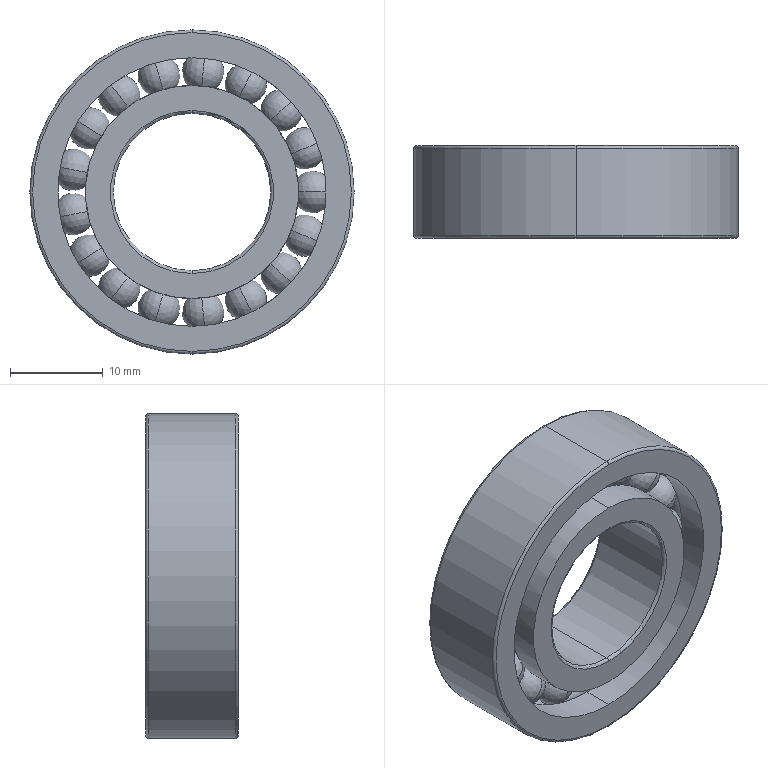Component | SolidWorks | -6003-1 | 1 solid | 112 faces | box 35 x 10 x 35 mm | volume 5427 mm3 | torus 62 | sphere 34 | cylinder 12 | plane 4 | commonest cylinder face diameters 29 x4 23 x4 35 x2 17 x2
build123d program:
from build123d import *

# Parameters (mm, degrees)
CIRCULAR_PATTERN1_COUNT = 17
FILLET1_R               = 0.3


with BuildPart() as part:
    # Sketch1 → Revolve1 (revolve)
    with BuildSketch(Plane.XY):
        with BuildLine():
            Line((-2.25, 13), (2.25, 13))
            ThreePointArc((2.25, 13), (0, 15.25), (-2.25, 13))
        make_face()
    revolve1 = revolve(axis=Axis((-4.597, 13, 0), (1, 0, 0)))

    # Sketch2 → Revolve2 (revolve)
    with BuildSketch(Plane.XY, mode=Mode.PRIVATE) as revolve2_sk:
        with BuildLine():
            Line((-5, 11.5), (-5, 8.5))
            Line((-5, 8.5), (5, 8.5))
            Line((5, 8.5), (5, 11.5))
            Line((5, 11.5), (1.664, 11.5))
            ThreePointArc((1.664, 11.5), (0, 10.76), (-1.664, 11.5))
            Line((-1.664, 11.5), (-5, 11.5))
        make_face()
    revolve(revolve2_sk.sketch.rotate(Axis((-6.971, 0, 0), (1, 0, 0)), 90), axis=Axis((-6.971, 0, 0), (1, 0, 0)))

    # Sketch3 → Revolve3 (revolve)
    with BuildSketch(Plane.XY, mode=Mode.PRIVATE) as revolve3_sk:
        with BuildLine():
            Line((-5, 17.5), (5, 17.5))
            Line((5, 17.5), (5, 14.5))
            Line((5, 14.5), (1.664, 14.5))
            ThreePointArc((1.664, 14.5), (0, 15.24), (-1.664, 14.5))
            Line((-1.664, 14.5), (-5, 14.5))
            Line((-5, 14.5), (-5, 17.5))
        make_face()
    revolve(revolve3_sk.sketch.rotate(Axis((-8.711, 0, 0), (1, 0, 0)), 90), axis=Axis((-8.711, 0, 0), (1, 0, 0)))

    # Circular-Pattern1: Revolve1 ×17 about axis
    circular_pattern1_axis = Axis((0, 0, 0), (1, 0, 0))
    for i in range(1, CIRCULAR_PATTERN1_COUNT):
        add(revolve1.rotate(circular_pattern1_axis, i * 360 / CIRCULAR_PATTERN1_COUNT))

    # Fillet1
    fillet1_edges = [part.edges().sort_by_distance(p)[0] for p in [
        (-5, 0, -17.5),
        (5, 0, -17.5),
        (-5, 0, -8.5),
        (5, 0, -8.5),
    ]]
    fillet(fillet1_edges, radius=FILLET1_R)


solid = part.part

# Placed as in the assembly
solid = solid.moved(Location((-29.507, 222.589, 458), (0, 0, -90)))